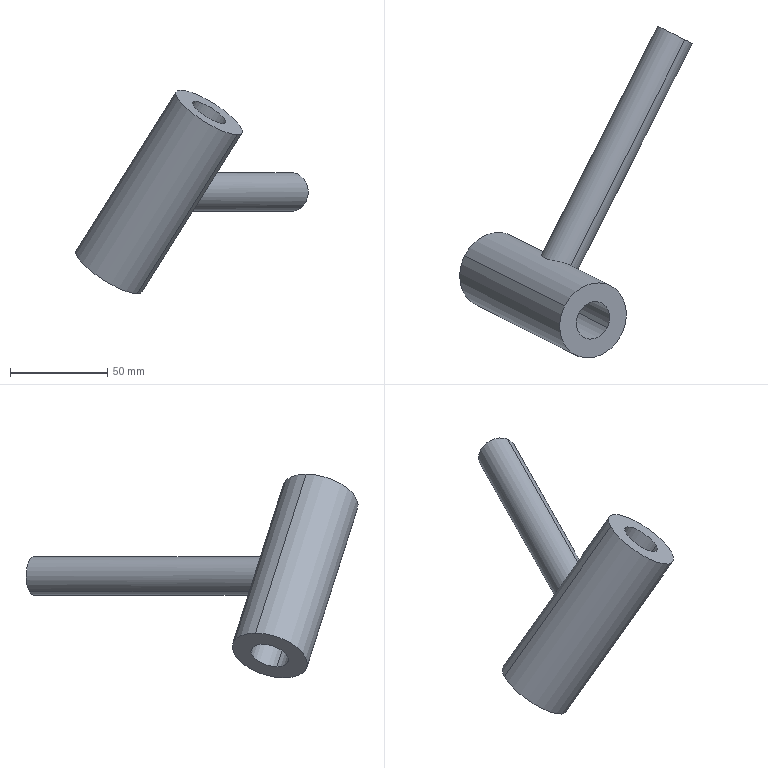Component | SolidWorks | Assembly4-1_Part26-1 | 2 solids | 10 faces | box 119.59 x 170.65 x 104.78 mm | volume 135292 mm3 | cylinder 7 | plane 3 | commonest cylinder face diameters 20 x4 40 x3
STEP:
#1=COLOUR_RGB('',0.7922,0.8196,0.9333);
#2=FILL_AREA_STYLE_COLOUR('',#1);
#3=FILL_AREA_STYLE('',(#2));
#4=SURFACE_STYLE_FILL_AREA(#3);
#5=SURFACE_SIDE_STYLE('',(#4));
#6=SURFACE_STYLE_USAGE(.BOTH.,#5);
#7=PRESENTATION_STYLE_ASSIGNMENT((#6));
#8=CARTESIAN_POINT('',(-16.069,-34.303,43.199));
#9=VERTEX_POINT('',#8);
#10=CARTESIAN_POINT('',(-16.474,-34.098,42.555));
#11=VERTEX_POINT('',#10);
#12=CARTESIAN_POINT('',(-16.272,-34.201,42.877));
#13=DIRECTION('',(0.4521,0.892,0.));
#14=DIRECTION('',(0.514,-0.2605,0.8172));
#15=AXIS2_PLACEMENT_3D('',#12,#13,#14);
#16=CIRCLE('',#15,0.3937);
#17=EDGE_CURVE('',#9,#11,#16,.T.);
#18=ORIENTED_EDGE('',*,*,#17,.F.);
#19=CARTESIAN_POINT('',(-18.383,-38.869,43.199));
#20=VERTEX_POINT('',#19);
#21=CARTESIAN_POINT('',(-16.069,-34.303,43.199));
#22=DIRECTION('',(-0.4521,-0.892,-0.));
#23=VECTOR('',#22,39.37);
#24=LINE('',#21,#23);
#25=EDGE_CURVE('',#9,#20,#24,.T.);
#26=ORIENTED_EDGE('',*,*,#25,.T.);
#27=CARTESIAN_POINT('',(-18.788,-38.664,42.555));
#28=VERTEX_POINT('',#27);
#29=CARTESIAN_POINT('',(-18.383,-38.869,43.199));
#30=CARTESIAN_POINT('',(-18.364,-38.878,43.184));
#31=CARTESIAN_POINT('',(-18.347,-38.889,43.167));
#32=CARTESIAN_POINT('',(-18.325,-38.904,43.138));
#33=CARTESIAN_POINT('',(-18.318,-38.909,43.128));
#34=CARTESIAN_POINT('',(-18.305,-38.92,43.108));
#35=CARTESIAN_POINT('',(-18.3,-38.925,43.097));
#36=CARTESIAN_POINT('',(-18.285,-38.941,43.064));
#37=CARTESIAN_POINT('',(-18.277,-38.951,43.041));
#38=CARTESIAN_POINT('',(-18.269,-38.965,43.005));
#39=CARTESIAN_POINT('',(-18.267,-38.97,42.993));
#40=CARTESIAN_POINT('',(-18.264,-38.979,42.969));
#41=CARTESIAN_POINT('',(-18.263,-38.983,42.956));
#42=CARTESIAN_POINT('',(-18.262,-38.991,42.931));
#43=CARTESIAN_POINT('',(-18.262,-38.995,42.919));
#44=CARTESIAN_POINT('',(-18.264,-39.002,42.894));
#45=CARTESIAN_POINT('',(-18.265,-39.005,42.881));
#46=CARTESIAN_POINT('',(-18.27,-39.013,42.842));
#47=CARTESIAN_POINT('',(-18.276,-39.017,42.817));
#48=CARTESIAN_POINT('',(-18.286,-39.02,42.78));
#49=CARTESIAN_POINT('',(-18.291,-39.021,42.767));
#50=CARTESIAN_POINT('',(-18.3,-39.021,42.743));
#51=CARTESIAN_POINT('',(-18.305,-39.02,42.73));
#52=CARTESIAN_POINT('',(-18.321,-39.017,42.695));
#53=CARTESIAN_POINT('',(-18.333,-39.013,42.672));
#54=CARTESIAN_POINT('',(-18.353,-39.002,42.64));
#55=CARTESIAN_POINT('',(-18.36,-38.998,42.629));
#56=CARTESIAN_POINT('',(-18.375,-38.989,42.609));
#57=CARTESIAN_POINT('',(-18.382,-38.984,42.6));
#58=CARTESIAN_POINT('',(-18.398,-38.973,42.582));
#59=CARTESIAN_POINT('',(-18.406,-38.967,42.574));
#60=CARTESIAN_POINT('',(-18.422,-38.954,42.558));
#61=CARTESIAN_POINT('',(-18.431,-38.947,42.55));
#62=CARTESIAN_POINT('',(-18.456,-38.925,42.53));
#63=CARTESIAN_POINT('',(-18.474,-38.91,42.518));
#64=CARTESIAN_POINT('',(-18.501,-38.885,42.505));
#65=CARTESIAN_POINT('',(-18.511,-38.876,42.501));
#66=CARTESIAN_POINT('',(-18.53,-38.859,42.494));
#67=CARTESIAN_POINT('',(-18.539,-38.85,42.491));
#68=CARTESIAN_POINT('',(-18.568,-38.825,42.485));
#69=CARTESIAN_POINT('',(-18.587,-38.807,42.483));
#70=CARTESIAN_POINT('',(-18.628,-38.773,42.484));
#71=CARTESIAN_POINT('',(-18.648,-38.756,42.487));
#72=CARTESIAN_POINT('',(-18.678,-38.733,42.495));
#73=CARTESIAN_POINT('',(-18.688,-38.726,42.499));
#74=CARTESIAN_POINT('',(-18.709,-38.711,42.507));
#75=CARTESIAN_POINT('',(-18.719,-38.704,42.512));
#76=CARTESIAN_POINT('',(-18.749,-38.685,42.527));
#77=CARTESIAN_POINT('',(-18.769,-38.673,42.54));
#78=CARTESIAN_POINT('',(-18.788,-38.664,42.555));
#79=B_SPLINE_CURVE_WITH_KNOTS('',3,(#29,#30,#31,#32,#33,#34,#35,#36,#37,#38,#39,#40,#41,#42,#43,#44,#45,#46,#47,#48,#49,#50,#51,#52,#53,#54,#55,#56,#57,#58,#59,#60,#61,#62,#63,#64,#65,#66,#67,#68,#69,#70,#71,#72,#73,#74,#75,#76,#77,#78),.UNSPECIFIED.,.F.,.F.,(4,2,2,2,2,2,2,2,2,2,2,2,2,2,2,2,2,2,2,2,2,2,2,2,4),(0.,0.001988,0.002982,0.003976,0.005964,0.006958,0.007952,0.008947,0.009941,0.01193,0.01292,0.01392,0.0159,0.0169,0.01789,0.01889,0.01988,0.02187,0.02286,0.02386,0.02585,0.02783,0.02883,0.02982,0.03181),.UNSPECIFIED.);
#80=EDGE_CURVE('',#20,#28,#79,.T.);
#81=ORIENTED_EDGE('',*,*,#80,.T.);
#82=CARTESIAN_POINT('',(-16.474,-34.098,42.555));
#83=DIRECTION('',(-0.4521,-0.892,-0.));
#84=VECTOR('',#83,39.37);
#85=LINE('',#82,#84);
#86=EDGE_CURVE('',#11,#28,#85,.T.);
#87=ORIENTED_EDGE('',*,*,#86,.F.);
#88=EDGE_LOOP('',(#18,#26,#81,#87));
#89=FACE_OUTER_BOUND('',#88,.T.);
#90=CARTESIAN_POINT('',(-16.272,-34.201,42.877));
#91=DIRECTION('',(-0.4521,-0.892,-0.));
#92=DIRECTION('',(-0.514,0.2605,-0.8172));
#93=AXIS2_PLACEMENT_3D('',#90,#91,#92);
#94=CYLINDRICAL_SURFACE('',#93,0.3937);
#95=ADVANCED_FACE('',(#89),#94,.T.);
#96=ORIENTED_EDGE('',*,*,#25,.F.);
#97=CARTESIAN_POINT('',(-16.272,-34.201,42.877));
#98=DIRECTION('',(0.4521,0.892,0.));
#99=DIRECTION('',(0.514,-0.2605,0.8172));
#100=AXIS2_PLACEMENT_3D('',#97,#98,#99);
#101=CIRCLE('',#100,0.3937);
#102=EDGE_CURVE('',#11,#9,#101,.T.);
#103=ORIENTED_EDGE('',*,*,#102,.F.);
#104=ORIENTED_EDGE('',*,*,#86,.T.);
#105=CARTESIAN_POINT('',(-18.788,-38.664,42.555));
#106=CARTESIAN_POINT('',(-18.807,-38.654,42.57));
#107=CARTESIAN_POINT('',(-18.826,-38.646,42.588));
#108=CARTESIAN_POINT('',(-18.86,-38.634,42.626));
#109=CARTESIAN_POINT('',(-18.876,-38.631,42.646));
#110=CARTESIAN_POINT('',(-18.904,-38.626,42.69));
#111=CARTESIAN_POINT('',(-18.917,-38.626,42.713));
#112=CARTESIAN_POINT('',(-18.933,-38.628,42.749));
#113=CARTESIAN_POINT('',(-18.938,-38.629,42.761));
#114=CARTESIAN_POINT('',(-18.947,-38.632,42.786));
#115=CARTESIAN_POINT('',(-18.951,-38.634,42.798));
#116=CARTESIAN_POINT('',(-18.962,-38.64,42.836));
#117=CARTESIAN_POINT('',(-18.966,-38.645,42.861));
#118=CARTESIAN_POINT('',(-18.97,-38.655,42.899));
#119=CARTESIAN_POINT('',(-18.971,-38.658,42.912));
#120=CARTESIAN_POINT('',(-18.971,-38.664,42.937));
#121=CARTESIAN_POINT('',(-18.97,-38.668,42.95));
#122=CARTESIAN_POINT('',(-18.966,-38.679,42.987));
#123=CARTESIAN_POINT('',(-18.961,-38.686,43.011));
#124=CARTESIAN_POINT('',(-18.949,-38.697,43.047));
#125=CARTESIAN_POINT('',(-18.944,-38.701,43.059));
#126=CARTESIAN_POINT('',(-18.933,-38.708,43.082));
#127=CARTESIAN_POINT('',(-18.921,-38.715,43.104));
#128=CARTESIAN_POINT('',(-18.907,-38.721,43.125));
#129=CARTESIAN_POINT('',(-18.891,-38.728,43.144));
#130=CARTESIAN_POINT('',(-18.882,-38.731,43.154));
#131=CARTESIAN_POINT('',(-18.855,-38.74,43.181));
#132=CARTESIAN_POINT('',(-18.834,-38.745,43.197));
#133=CARTESIAN_POINT('',(-18.802,-38.753,43.217));
#134=CARTESIAN_POINT('',(-18.79,-38.756,43.224));
#135=CARTESIAN_POINT('',(-18.767,-38.761,43.235));
#136=CARTESIAN_POINT('',(-18.755,-38.763,43.24));
#137=CARTESIAN_POINT('',(-18.731,-38.768,43.249));
#138=CARTESIAN_POINT('',(-18.719,-38.771,43.253));
#139=CARTESIAN_POINT('',(-18.694,-38.776,43.26));
#140=CARTESIAN_POINT('',(-18.682,-38.778,43.263));
#141=CARTESIAN_POINT('',(-18.643,-38.786,43.269));
#142=CARTESIAN_POINT('',(-18.618,-38.792,43.271));
#143=CARTESIAN_POINT('',(-18.58,-38.801,43.271));
#144=CARTESIAN_POINT('',(-18.567,-38.804,43.27));
#145=CARTESIAN_POINT('',(-18.542,-38.811,43.267));
#146=CARTESIAN_POINT('',(-18.529,-38.814,43.264));
#147=CARTESIAN_POINT('',(-18.492,-38.825,43.256));
#148=CARTESIAN_POINT('',(-18.469,-38.833,43.248));
#149=CARTESIAN_POINT('',(-18.435,-38.845,43.232));
#150=CARTESIAN_POINT('',(-18.424,-38.85,43.227));
#151=CARTESIAN_POINT('',(-18.403,-38.859,43.214));
#152=CARTESIAN_POINT('',(-18.393,-38.864,43.207));
#153=CARTESIAN_POINT('',(-18.383,-38.869,43.199));
#154=B_SPLINE_CURVE_WITH_KNOTS('',3,(#105,#106,#107,#108,#109,#110,#111,#112,#113,#114,#115,#116,#117,#118,#119,#120,#121,#122,#123,#124,#125,#126,#127,#128,#129,#130,#131,#132,#133,#134,#135,#136,#137,#138,#139,#140,#141,#142,#143,#144,#145,#146,#147,#148,#149,#150,#151,#152,#153),.UNSPECIFIED.,.F.,.F.,(4,2,2,2,2,2,2,2,2,2,2,1,2,2,2,2,2,2,2,2,2,2,2,2,4),(0.03181,0.03379,0.03578,0.03776,0.03876,0.03975,0.04173,0.04273,0.04372,0.0457,0.04669,0.04769,0.04868,0.04967,0.05166,0.05265,0.05364,0.05463,0.05563,0.05761,0.0586,0.05959,0.06158,0.06257,0.06356),.UNSPECIFIED.);
#155=EDGE_CURVE('',#28,#20,#154,.T.);
#156=ORIENTED_EDGE('',*,*,#155,.T.);
#157=EDGE_LOOP('',(#96,#103,#104,#156));
#158=FACE_OUTER_BOUND('',#157,.T.);
#159=CARTESIAN_POINT('',(-16.272,-34.201,42.877));
#160=DIRECTION('',(-0.4521,-0.892,-0.));
#161=DIRECTION('',(-0.514,0.2605,-0.8172));
#162=AXIS2_PLACEMENT_3D('',#159,#160,#161);
#163=CYLINDRICAL_SURFACE('',#162,0.3937);
#164=ADVANCED_FACE('',(#158),#163,.T.);
#165=ORIENTED_EDGE('',*,*,#102,.T.);
#166=ORIENTED_EDGE('',*,*,#17,.T.);
#167=EDGE_LOOP('',(#165,#166));
#168=FACE_OUTER_BOUND('',#167,.T.);
#169=CARTESIAN_POINT('',(-16.272,-34.201,42.877));
#170=DIRECTION('',(0.4521,0.892,0.));
#171=DIRECTION('',(0.514,-0.2605,0.8172));
#172=AXIS2_PLACEMENT_3D('',#169,#170,#171);
#173=PLANE('',#172);
#174=ADVANCED_FACE('',(#168),#173,.T.);
#175=ORIENTED_EDGE('',*,*,#155,.F.);
#176=ORIENTED_EDGE('',*,*,#80,.F.);
#177=EDGE_LOOP('',(#175,#176));
#178=FACE_OUTER_BOUND('',#177,.T.);
#179=CARTESIAN_POINT('',(-19.953,-38.956,41.268));
#180=DIRECTION('',(0.514,-0.2605,0.8172));
#181=DIRECTION('',(-0.729,0.3695,0.5763));
#182=AXIS2_PLACEMENT_3D('',#179,#180,#181);
#183=CYLINDRICAL_SURFACE('',#182,0.7874);
#184=ADVANCED_FACE('',(#178),#183,.F.);
#185=CLOSED_SHELL('',(#95,#164,#174,#184));
#186=MANIFOLD_SOLID_BREP('',#185);
#187=STYLED_ITEM('',(#7),#186);
#188=PRESENTATION_LAYER_ASSIGNMENT('','',(#187));
#189=(LENGTH_UNIT()NAMED_UNIT(*)SI_UNIT($,.METRE.));
#190=LENGTH_MEASURE_WITH_UNIT(LENGTH_MEASURE(0.0254),#189);
#191=DIMENSIONAL_EXPONENTS(1.,0.,0.,0.,0.,0.,0.);
#192=(CONVERSION_BASED_UNIT('',#190)LENGTH_UNIT()NAMED_UNIT(#191));
#193=UNCERTAINTY_MEASURE_WITH_UNIT(LENGTH_MEASURE(0.00001),#192,'','');
#194=(NAMED_UNIT(*)PLANE_ANGLE_UNIT()SI_UNIT($,.RADIAN.));
#195=(NAMED_UNIT(*)SI_UNIT($,.STERADIAN.)SOLID_ANGLE_UNIT());
#196=(GEOMETRIC_REPRESENTATION_CONTEXT(3)GLOBAL_UNCERTAINTY_ASSIGNED_CONTEXT((#193))GLOBAL_UNIT_ASSIGNED_CONTEXT((#192,#194,#195))REPRESENTATION_CONTEXT('',''));
#197=MECHANICAL_DESIGN_GEOMETRIC_PRESENTATION_REPRESENTATION('',(#187),#196);
#198=CARTESIAN_POINT('',(-20.24,-38.81,41.495));
#199=VERTEX_POINT('',#198);
#200=CARTESIAN_POINT('',(-19.666,-39.101,41.042));
#201=VERTEX_POINT('',#200);
#202=CARTESIAN_POINT('',(-19.953,-38.956,41.268));
#203=DIRECTION('',(-0.514,0.2605,-0.8172));
#204=DIRECTION('',(0.729,-0.3695,-0.5763));
#205=AXIS2_PLACEMENT_3D('',#202,#203,#204);
#206=CIRCLE('',#205,0.3937);
#207=EDGE_CURVE('',#199,#201,#206,.T.);
#208=ORIENTED_EDGE('',*,*,#207,.T.);
#209=CARTESIAN_POINT('',(-17.643,-40.127,44.259));
#210=VERTEX_POINT('',#209);
#211=CARTESIAN_POINT('',(-19.666,-39.101,41.042));
#212=DIRECTION('',(0.514,-0.2605,0.8172));
#213=VECTOR('',#212,39.37);
#214=LINE('',#211,#213);
#215=EDGE_CURVE('',#201,#210,#214,.T.);
#216=ORIENTED_EDGE('',*,*,#215,.T.);
#217=CARTESIAN_POINT('',(-18.217,-39.836,44.713));
#218=VERTEX_POINT('',#217);
#219=CARTESIAN_POINT('',(-17.93,-39.981,44.486));
#220=DIRECTION('',(-0.514,0.2605,-0.8172));
#221=DIRECTION('',(0.729,-0.3695,-0.5763));
#222=AXIS2_PLACEMENT_3D('',#219,#220,#221);
#223=CIRCLE('',#222,0.3937);
#224=EDGE_CURVE('',#218,#210,#223,.T.);
#225=ORIENTED_EDGE('',*,*,#224,.F.);
#226=CARTESIAN_POINT('',(-20.24,-38.81,41.495));
#227=DIRECTION('',(0.514,-0.2605,0.8172));
#228=VECTOR('',#227,39.37);
#229=LINE('',#226,#228);
#230=EDGE_CURVE('',#199,#218,#229,.T.);
#231=ORIENTED_EDGE('',*,*,#230,.F.);
#232=EDGE_LOOP('',(#208,#216,#225,#231));
#233=FACE_OUTER_BOUND('',#232,.T.);
#234=CARTESIAN_POINT('',(-19.953,-38.956,41.268));
#235=DIRECTION('',(0.514,-0.2605,0.8172));
#236=DIRECTION('',(-0.729,0.3695,0.5763));
#237=AXIS2_PLACEMENT_3D('',#234,#235,#236);
#238=CYLINDRICAL_SURFACE('',#237,0.3937);
#239=ADVANCED_FACE('',(#233),#238,.F.);
#240=CARTESIAN_POINT('',(-19.379,-39.246,40.815));
#241=VERTEX_POINT('',#240);
#242=CARTESIAN_POINT('',(-20.527,-38.665,41.722));
#243=VERTEX_POINT('',#242);
#244=CARTESIAN_POINT('',(-19.953,-38.956,41.268));
#245=DIRECTION('',(-0.514,0.2605,-0.8172));
#246=DIRECTION('',(0.729,-0.3695,-0.5763));
#247=AXIS2_PLACEMENT_3D('',#244,#245,#246);
#248=CIRCLE('',#247,0.7874);
#249=EDGE_CURVE('',#241,#243,#248,.T.);
#250=ORIENTED_EDGE('',*,*,#249,.F.);
#251=CARTESIAN_POINT('',(-17.356,-40.272,44.032));
#252=VERTEX_POINT('',#251);
#253=CARTESIAN_POINT('',(-19.379,-39.246,40.815));
#254=DIRECTION('',(0.514,-0.2605,0.8172));
#255=VECTOR('',#254,39.37);
#256=LINE('',#253,#255);
#257=EDGE_CURVE('',#241,#252,#256,.T.);
#258=ORIENTED_EDGE('',*,*,#257,.T.);
#259=CARTESIAN_POINT('',(-18.504,-39.69,44.94));
#260=VERTEX_POINT('',#259);
#261=CARTESIAN_POINT('',(-17.93,-39.981,44.486));
#262=DIRECTION('',(-0.514,0.2605,-0.8172));
#263=DIRECTION('',(0.729,-0.3695,-0.5763));
#264=AXIS2_PLACEMENT_3D('',#261,#262,#263);
#265=CIRCLE('',#264,0.7874);
#266=EDGE_CURVE('',#252,#260,#265,.T.);
#267=ORIENTED_EDGE('',*,*,#266,.T.);
#268=CARTESIAN_POINT('',(-20.527,-38.665,41.722));
#269=DIRECTION('',(0.514,-0.2605,0.8172));
#270=VECTOR('',#269,39.37);
#271=LINE('',#268,#270);
#272=EDGE_CURVE('',#243,#260,#271,.T.);
#273=ORIENTED_EDGE('',*,*,#272,.F.);
#274=EDGE_LOOP('',(#250,#258,#267,#273));
#275=FACE_OUTER_BOUND('',#274,.T.);
#276=CARTESIAN_POINT('',(-19.953,-38.956,41.268));
#277=DIRECTION('',(0.514,-0.2605,0.8172));
#278=DIRECTION('',(-0.729,0.3695,0.5763));
#279=AXIS2_PLACEMENT_3D('',#276,#277,#278);
#280=CYLINDRICAL_SURFACE('',#279,0.7874);
#281=ADVANCED_FACE('',(#275),#280,.T.);
#282=CARTESIAN_POINT('',(-19.953,-38.956,41.268));
#283=DIRECTION('',(-0.514,0.2605,-0.8172));
#284=DIRECTION('',(0.729,-0.3695,-0.5763));
#285=AXIS2_PLACEMENT_3D('',#282,#283,#284);
#286=CIRCLE('',#285,0.7874);
#287=EDGE_CURVE('',#243,#241,#286,.T.);
#288=ORIENTED_EDGE('',*,*,#287,.T.);
#289=ORIENTED_EDGE('',*,*,#249,.T.);
#290=EDGE_LOOP('',(#288,#289));
#291=FACE_OUTER_BOUND('',#290,.T.);
#292=ORIENTED_EDGE('',*,*,#207,.F.);
#293=CARTESIAN_POINT('',(-19.953,-38.956,41.268));
#294=DIRECTION('',(-0.514,0.2605,-0.8172));
#295=DIRECTION('',(0.729,-0.3695,-0.5763));
#296=AXIS2_PLACEMENT_3D('',#293,#294,#295);
#297=CIRCLE('',#296,0.3937);
#298=EDGE_CURVE('',#201,#199,#297,.T.);
#299=ORIENTED_EDGE('',*,*,#298,.F.);
#300=EDGE_LOOP('',(#292,#299));
#301=FACE_BOUND('',#300,.T.);
#302=CARTESIAN_POINT('',(-19.953,-38.956,41.268));
#303=DIRECTION('',(-0.514,0.2605,-0.8172));
#304=DIRECTION('',(0.729,-0.3695,-0.5763));
#305=AXIS2_PLACEMENT_3D('',#302,#303,#304);
#306=PLANE('',#305);
#307=ADVANCED_FACE('',(#291,#301),#306,.T.);
#308=CARTESIAN_POINT('',(-17.93,-39.981,44.486));
#309=DIRECTION('',(-0.514,0.2605,-0.8172));
#310=DIRECTION('',(0.729,-0.3695,-0.5763));
#311=AXIS2_PLACEMENT_3D('',#308,#309,#310);
#312=CIRCLE('',#311,0.7874);
#313=EDGE_CURVE('',#260,#252,#312,.T.);
#314=ORIENTED_EDGE('',*,*,#313,.F.);
#315=ORIENTED_EDGE('',*,*,#266,.F.);
#316=EDGE_LOOP('',(#314,#315));
#317=FACE_OUTER_BOUND('',#316,.T.);
#318=ORIENTED_EDGE('',*,*,#224,.T.);
#319=CARTESIAN_POINT('',(-17.93,-39.981,44.486));
#320=DIRECTION('',(-0.514,0.2605,-0.8172));
#321=DIRECTION('',(0.729,-0.3695,-0.5763));
#322=AXIS2_PLACEMENT_3D('',#319,#320,#321);
#323=CIRCLE('',#322,0.3937);
#324=EDGE_CURVE('',#210,#218,#323,.T.);
#325=ORIENTED_EDGE('',*,*,#324,.T.);
#326=EDGE_LOOP('',(#318,#325));
#327=FACE_BOUND('',#326,.T.);
#328=CARTESIAN_POINT('',(-17.93,-39.981,44.486));
#329=DIRECTION('',(-0.514,0.2605,-0.8172));
#330=DIRECTION('',(0.729,-0.3695,-0.5763));
#331=AXIS2_PLACEMENT_3D('',#328,#329,#330);
#332=PLANE('',#331);
#333=ADVANCED_FACE('',(#317,#327),#332,.F.);
#334=ORIENTED_EDGE('',*,*,#257,.F.);
#335=ORIENTED_EDGE('',*,*,#287,.F.);
#336=ORIENTED_EDGE('',*,*,#272,.T.);
#337=ORIENTED_EDGE('',*,*,#313,.T.);
#338=EDGE_LOOP('',(#334,#335,#336,#337));
#339=FACE_OUTER_BOUND('',#338,.T.);
#340=CARTESIAN_POINT('',(-19.953,-38.956,41.268));
#341=DIRECTION('',(0.514,-0.2605,0.8172));
#342=DIRECTION('',(-0.729,0.3695,0.5763));
#343=AXIS2_PLACEMENT_3D('',#340,#341,#342);
#344=CYLINDRICAL_SURFACE('',#343,0.7874);
#345=ADVANCED_FACE('',(#339),#344,.T.);
#346=ORIENTED_EDGE('',*,*,#215,.F.);
#347=ORIENTED_EDGE('',*,*,#298,.T.);
#348=ORIENTED_EDGE('',*,*,#230,.T.);
#349=ORIENTED_EDGE('',*,*,#324,.F.);
#350=EDGE_LOOP('',(#346,#347,#348,#349));
#351=FACE_OUTER_BOUND('',#350,.T.);
#352=CARTESIAN_POINT('',(-19.953,-38.956,41.268));
#353=DIRECTION('',(0.514,-0.2605,0.8172));
#354=DIRECTION('',(-0.729,0.3695,0.5763));
#355=AXIS2_PLACEMENT_3D('',#352,#353,#354);
#356=CYLINDRICAL_SURFACE('',#355,0.3937);
#357=ADVANCED_FACE('',(#351),#356,.F.);
#358=CLOSED_SHELL('',(#239,#281,#307,#333,#345,#357));
#359=MANIFOLD_SOLID_BREP('',#358);
#360=CARTESIAN_POINT('',(0.,0.,0.));
#361=DIRECTION('',(0.,0.,1.));
#362=DIRECTION('',(1.,0.,0.));
#363=AXIS2_PLACEMENT_3D('',#360,#361,#362);
#364=(LENGTH_UNIT()NAMED_UNIT(*)SI_UNIT($,.METRE.));
#365=LENGTH_MEASURE_WITH_UNIT(LENGTH_MEASURE(0.0254),#364);
#366=DIMENSIONAL_EXPONENTS(1.,0.,0.,0.,0.,0.,0.);
#367=(CONVERSION_BASED_UNIT('',#365)LENGTH_UNIT()NAMED_UNIT(#366));
#368=UNCERTAINTY_MEASURE_WITH_UNIT(LENGTH_MEASURE(0.00001),#367,'','');
#369=(NAMED_UNIT(*)PLANE_ANGLE_UNIT()SI_UNIT($,.RADIAN.));
#370=(NAMED_UNIT(*)SI_UNIT($,.STERADIAN.)SOLID_ANGLE_UNIT());
#371=(GEOMETRIC_REPRESENTATION_CONTEXT(3)GLOBAL_UNCERTAINTY_ASSIGNED_CONTEXT((#368))GLOBAL_UNIT_ASSIGNED_CONTEXT((#367,#369,#370))REPRESENTATION_CONTEXT('',''));
#372=ADVANCED_BREP_SHAPE_REPRESENTATION('',(#186,#359,#363),#371);
#373=COLOUR_RGB('',0.7922,0.8196,0.9333);
#374=FILL_AREA_STYLE_COLOUR('',#373);
#375=FILL_AREA_STYLE('',(#374));
#376=SURFACE_STYLE_FILL_AREA(#375);
#377=SURFACE_SIDE_STYLE('',(#376));
#378=SURFACE_STYLE_USAGE(.BOTH.,#377);
#379=PRESENTATION_STYLE_ASSIGNMENT((#378));
#380=STYLED_ITEM('',(#379),#359);
#381=PRESENTATION_LAYER_ASSIGNMENT('','',(#380));
#382=(LENGTH_UNIT()NAMED_UNIT(*)SI_UNIT($,.METRE.));
#383=LENGTH_MEASURE_WITH_UNIT(LENGTH_MEASURE(0.0254),#382);
#384=DIMENSIONAL_EXPONENTS(1.,0.,0.,0.,0.,0.,0.);
#385=(CONVERSION_BASED_UNIT('',#383)LENGTH_UNIT()NAMED_UNIT(#384));
#386=UNCERTAINTY_MEASURE_WITH_UNIT(LENGTH_MEASURE(0.00001),#385,'','');
#387=(NAMED_UNIT(*)PLANE_ANGLE_UNIT()SI_UNIT($,.RADIAN.));
#388=(NAMED_UNIT(*)SI_UNIT($,.STERADIAN.)SOLID_ANGLE_UNIT());
#389=(GEOMETRIC_REPRESENTATION_CONTEXT(3)GLOBAL_UNCERTAINTY_ASSIGNED_CONTEXT((#386))GLOBAL_UNIT_ASSIGNED_CONTEXT((#385,#387,#388))REPRESENTATION_CONTEXT('',''));
#390=MECHANICAL_DESIGN_GEOMETRIC_PRESENTATION_REPRESENTATION('',(#380),#389);